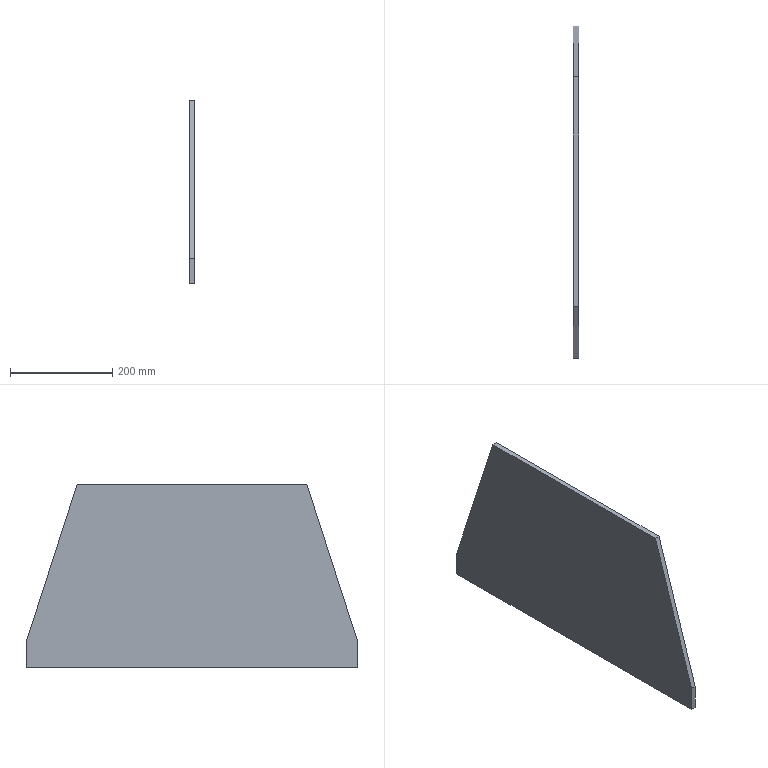Component | SolidWorks | Main-1_650X450X360X10-1 | 1 solid | 8 faces | box 10 x 650 x 360 mm | volume 2030000 mm3 | plane 8 | material Plain Carbon Steel
STEP:
#1=CARTESIAN_POINT('',(-132.764,88.438,207.322));
#2=VERTEX_POINT('',#1);
#3=CARTESIAN_POINT('',(-132.764,84.501,219.527));
#4=VERTEX_POINT('',#3);
#5=CARTESIAN_POINT('',(-132.764,84.501,219.527));
#6=DIRECTION('',(0.,-0.307,0.9517));
#7=VECTOR('',#6,39.37);
#8=LINE('',#5,#7);
#9=EDGE_CURVE('',#2,#4,#8,.T.);
#10=ORIENTED_EDGE('',*,*,#9,.F.);
#11=CARTESIAN_POINT('',(-133.157,88.438,207.322));
#12=VERTEX_POINT('',#11);
#13=CARTESIAN_POINT('',(-133.157,88.438,207.322));
#14=DIRECTION('',(1.,0.,-0.));
#15=VECTOR('',#14,39.37);
#16=LINE('',#13,#15);
#17=EDGE_CURVE('',#12,#2,#16,.T.);
#18=ORIENTED_EDGE('',*,*,#17,.F.);
#19=CARTESIAN_POINT('',(-133.157,84.501,219.527));
#20=VERTEX_POINT('',#19);
#21=CARTESIAN_POINT('',(-133.157,84.501,219.527));
#22=DIRECTION('',(0.,-0.307,0.9517));
#23=VECTOR('',#22,39.37);
#24=LINE('',#21,#23);
#25=EDGE_CURVE('',#12,#20,#24,.T.);
#26=ORIENTED_EDGE('',*,*,#25,.T.);
#27=CARTESIAN_POINT('',(-133.157,84.501,219.527));
#28=DIRECTION('',(1.,0.,-0.));
#29=VECTOR('',#28,39.37);
#30=LINE('',#27,#29);
#31=EDGE_CURVE('',#20,#4,#30,.T.);
#32=ORIENTED_EDGE('',*,*,#31,.T.);
#33=EDGE_LOOP('',(#10,#18,#26,#32));
#34=FACE_OUTER_BOUND('',#33,.T.);
#35=CARTESIAN_POINT('',(-133.157,84.501,219.527));
#36=DIRECTION('',(-0.,0.9517,0.307));
#37=DIRECTION('',(0.,-0.307,0.9517));
#38=AXIS2_PLACEMENT_3D('',#35,#36,#37);
#39=PLANE('',#38);
#40=ADVANCED_FACE('',(#34),#39,.T.);
#41=CARTESIAN_POINT('',(-132.764,88.438,205.353));
#42=VERTEX_POINT('',#41);
#43=CARTESIAN_POINT('',(-132.764,88.438,207.322));
#44=DIRECTION('',(0.,-0.,1.));
#45=VECTOR('',#44,39.37);
#46=LINE('',#43,#45);
#47=EDGE_CURVE('',#42,#2,#46,.T.);
#48=ORIENTED_EDGE('',*,*,#47,.F.);
#49=CARTESIAN_POINT('',(-133.157,88.438,205.353));
#50=VERTEX_POINT('',#49);
#51=CARTESIAN_POINT('',(-133.157,88.438,205.353));
#52=DIRECTION('',(1.,0.,-0.));
#53=VECTOR('',#52,39.37);
#54=LINE('',#51,#53);
#55=EDGE_CURVE('',#50,#42,#54,.T.);
#56=ORIENTED_EDGE('',*,*,#55,.F.);
#57=CARTESIAN_POINT('',(-133.157,88.438,207.322));
#58=DIRECTION('',(0.,-0.,1.));
#59=VECTOR('',#58,39.37);
#60=LINE('',#57,#59);
#61=EDGE_CURVE('',#50,#12,#60,.T.);
#62=ORIENTED_EDGE('',*,*,#61,.T.);
#63=ORIENTED_EDGE('',*,*,#17,.T.);
#64=EDGE_LOOP('',(#48,#56,#62,#63));
#65=FACE_OUTER_BOUND('',#64,.T.);
#66=CARTESIAN_POINT('',(-133.157,88.438,207.322));
#67=DIRECTION('',(-0.,1.,0.));
#68=DIRECTION('',(0.,-0.,1.));
#69=AXIS2_PLACEMENT_3D('',#66,#67,#68);
#70=PLANE('',#69);
#71=ADVANCED_FACE('',(#65),#70,.T.);
#72=CARTESIAN_POINT('',(-132.764,62.847,205.353));
#73=VERTEX_POINT('',#72);
#74=CARTESIAN_POINT('',(-132.764,88.438,205.353));
#75=DIRECTION('',(-0.,1.,0.));
#76=VECTOR('',#75,39.37);
#77=LINE('',#74,#76);
#78=EDGE_CURVE('',#73,#42,#77,.T.);
#79=ORIENTED_EDGE('',*,*,#78,.F.);
#80=CARTESIAN_POINT('',(-133.157,62.847,205.353));
#81=VERTEX_POINT('',#80);
#82=CARTESIAN_POINT('',(-133.157,62.847,205.353));
#83=DIRECTION('',(1.,0.,-0.));
#84=VECTOR('',#83,39.37);
#85=LINE('',#82,#84);
#86=EDGE_CURVE('',#81,#73,#85,.T.);
#87=ORIENTED_EDGE('',*,*,#86,.F.);
#88=CARTESIAN_POINT('',(-133.157,88.438,205.353));
#89=DIRECTION('',(-0.,1.,0.));
#90=VECTOR('',#89,39.37);
#91=LINE('',#88,#90);
#92=EDGE_CURVE('',#81,#50,#91,.T.);
#93=ORIENTED_EDGE('',*,*,#92,.T.);
#94=ORIENTED_EDGE('',*,*,#55,.T.);
#95=EDGE_LOOP('',(#79,#87,#93,#94));
#96=FACE_OUTER_BOUND('',#95,.T.);
#97=CARTESIAN_POINT('',(-133.157,88.438,205.353));
#98=DIRECTION('',(-0.,0.,-1.));
#99=DIRECTION('',(-0.,1.,0.));
#100=AXIS2_PLACEMENT_3D('',#97,#98,#99);
#101=PLANE('',#100);
#102=ADVANCED_FACE('',(#96),#101,.T.);
#103=CARTESIAN_POINT('',(-132.764,62.847,207.322));
#104=VERTEX_POINT('',#103);
#105=CARTESIAN_POINT('',(-132.764,62.847,205.353));
#106=DIRECTION('',(-0.,0.,-1.));
#107=VECTOR('',#106,39.37);
#108=LINE('',#105,#107);
#109=EDGE_CURVE('',#104,#73,#108,.T.);
#110=ORIENTED_EDGE('',*,*,#109,.F.);
#111=CARTESIAN_POINT('',(-133.157,62.847,207.322));
#112=VERTEX_POINT('',#111);
#113=CARTESIAN_POINT('',(-133.157,62.847,207.322));
#114=DIRECTION('',(1.,0.,-0.));
#115=VECTOR('',#114,39.37);
#116=LINE('',#113,#115);
#117=EDGE_CURVE('',#112,#104,#116,.T.);
#118=ORIENTED_EDGE('',*,*,#117,.F.);
#119=CARTESIAN_POINT('',(-133.157,62.847,205.353));
#120=DIRECTION('',(-0.,0.,-1.));
#121=VECTOR('',#120,39.37);
#122=LINE('',#119,#121);
#123=EDGE_CURVE('',#112,#81,#122,.T.);
#124=ORIENTED_EDGE('',*,*,#123,.T.);
#125=ORIENTED_EDGE('',*,*,#86,.T.);
#126=EDGE_LOOP('',(#110,#118,#124,#125));
#127=FACE_OUTER_BOUND('',#126,.T.);
#128=CARTESIAN_POINT('',(-133.157,62.847,205.353));
#129=DIRECTION('',(0.,-1.,-0.));
#130=DIRECTION('',(-0.,0.,-1.));
#131=AXIS2_PLACEMENT_3D('',#128,#129,#130);
#132=PLANE('',#131);
#133=ADVANCED_FACE('',(#127),#132,.T.);
#134=CARTESIAN_POINT('',(-132.764,66.784,219.527));
#135=VERTEX_POINT('',#134);
#136=CARTESIAN_POINT('',(-132.764,62.847,207.322));
#137=DIRECTION('',(-0.,-0.307,-0.9517));
#138=VECTOR('',#137,39.37);
#139=LINE('',#136,#138);
#140=EDGE_CURVE('',#135,#104,#139,.T.);
#141=ORIENTED_EDGE('',*,*,#140,.F.);
#142=CARTESIAN_POINT('',(-133.157,66.784,219.527));
#143=VERTEX_POINT('',#142);
#144=CARTESIAN_POINT('',(-133.157,66.784,219.527));
#145=DIRECTION('',(1.,0.,-0.));
#146=VECTOR('',#145,39.37);
#147=LINE('',#144,#146);
#148=EDGE_CURVE('',#143,#135,#147,.T.);
#149=ORIENTED_EDGE('',*,*,#148,.F.);
#150=CARTESIAN_POINT('',(-133.157,62.847,207.322));
#151=DIRECTION('',(-0.,-0.307,-0.9517));
#152=VECTOR('',#151,39.37);
#153=LINE('',#150,#152);
#154=EDGE_CURVE('',#143,#112,#153,.T.);
#155=ORIENTED_EDGE('',*,*,#154,.T.);
#156=ORIENTED_EDGE('',*,*,#117,.T.);
#157=EDGE_LOOP('',(#141,#149,#155,#156));
#158=FACE_OUTER_BOUND('',#157,.T.);
#159=CARTESIAN_POINT('',(-133.157,62.847,207.322));
#160=DIRECTION('',(0.,-0.9517,0.307));
#161=DIRECTION('',(-0.,-0.307,-0.9517));
#162=AXIS2_PLACEMENT_3D('',#159,#160,#161);
#163=PLANE('',#162);
#164=ADVANCED_FACE('',(#158),#163,.T.);
#165=CARTESIAN_POINT('',(-132.764,66.784,219.527));
#166=DIRECTION('',(0.,-1.,-0.));
#167=VECTOR('',#166,39.37);
#168=LINE('',#165,#167);
#169=EDGE_CURVE('',#4,#135,#168,.T.);
#170=ORIENTED_EDGE('',*,*,#169,.F.);
#171=ORIENTED_EDGE('',*,*,#31,.F.);
#172=CARTESIAN_POINT('',(-133.157,66.784,219.527));
#173=DIRECTION('',(0.,-1.,-0.));
#174=VECTOR('',#173,39.37);
#175=LINE('',#172,#174);
#176=EDGE_CURVE('',#20,#143,#175,.T.);
#177=ORIENTED_EDGE('',*,*,#176,.T.);
#178=ORIENTED_EDGE('',*,*,#148,.T.);
#179=EDGE_LOOP('',(#170,#171,#177,#178));
#180=FACE_OUTER_BOUND('',#179,.T.);
#181=CARTESIAN_POINT('',(-133.157,66.784,219.527));
#182=DIRECTION('',(0.,-0.,1.));
#183=DIRECTION('',(0.,-1.,-0.));
#184=AXIS2_PLACEMENT_3D('',#181,#182,#183);
#185=PLANE('',#184);
#186=ADVANCED_FACE('',(#180),#185,.T.);
#187=ORIENTED_EDGE('',*,*,#25,.F.);
#188=ORIENTED_EDGE('',*,*,#61,.F.);
#189=ORIENTED_EDGE('',*,*,#92,.F.);
#190=ORIENTED_EDGE('',*,*,#123,.F.);
#191=ORIENTED_EDGE('',*,*,#154,.F.);
#192=ORIENTED_EDGE('',*,*,#176,.F.);
#193=EDGE_LOOP('',(#187,#188,#189,#190,#191,#192));
#194=FACE_OUTER_BOUND('',#193,.T.);
#195=CARTESIAN_POINT('',(-133.157,62.847,219.527));
#196=DIRECTION('',(-1.,-0.,0.));
#197=DIRECTION('',(0.,-0.,1.));
#198=AXIS2_PLACEMENT_3D('',#195,#196,#197);
#199=PLANE('',#198);
#200=ADVANCED_FACE('',(#194),#199,.T.);
#201=ORIENTED_EDGE('',*,*,#9,.T.);
#202=ORIENTED_EDGE('',*,*,#169,.T.);
#203=ORIENTED_EDGE('',*,*,#140,.T.);
#204=ORIENTED_EDGE('',*,*,#109,.T.);
#205=ORIENTED_EDGE('',*,*,#78,.T.);
#206=ORIENTED_EDGE('',*,*,#47,.T.);
#207=EDGE_LOOP('',(#201,#202,#203,#204,#205,#206));
#208=FACE_OUTER_BOUND('',#207,.T.);
#209=CARTESIAN_POINT('',(-132.764,62.847,219.527));
#210=DIRECTION('',(-1.,-0.,0.));
#211=DIRECTION('',(0.,-0.,1.));
#212=AXIS2_PLACEMENT_3D('',#209,#210,#211);
#213=PLANE('',#212);
#214=ADVANCED_FACE('',(#208),#213,.F.);
#215=CLOSED_SHELL('',(#40,#71,#102,#133,#164,#186,#200,#214));
#216=MANIFOLD_SOLID_BREP('',#215);
#217=CARTESIAN_POINT('',(0.,0.,0.));
#218=DIRECTION('',(0.,0.,1.));
#219=DIRECTION('',(1.,0.,0.));
#220=AXIS2_PLACEMENT_3D('',#217,#218,#219);
#221=(LENGTH_UNIT()NAMED_UNIT(*)SI_UNIT($,.METRE.));
#222=LENGTH_MEASURE_WITH_UNIT(LENGTH_MEASURE(0.0254),#221);
#223=DIMENSIONAL_EXPONENTS(1.,0.,0.,0.,0.,0.,0.);
#224=(CONVERSION_BASED_UNIT('',#222)LENGTH_UNIT()NAMED_UNIT(#223));
#225=UNCERTAINTY_MEASURE_WITH_UNIT(LENGTH_MEASURE(0.00001),#224,'','');
#226=(NAMED_UNIT(*)PLANE_ANGLE_UNIT()SI_UNIT($,.RADIAN.));
#227=(NAMED_UNIT(*)SI_UNIT($,.STERADIAN.)SOLID_ANGLE_UNIT());
#228=(GEOMETRIC_REPRESENTATION_CONTEXT(3)GLOBAL_UNCERTAINTY_ASSIGNED_CONTEXT((#225))GLOBAL_UNIT_ASSIGNED_CONTEXT((#224,#226,#227))REPRESENTATION_CONTEXT('',''));
#229=ADVANCED_BREP_SHAPE_REPRESENTATION('',(#216,#220),#228);
#230=COLOUR_RGB('',0.7922,0.8196,0.9333);
#231=FILL_AREA_STYLE_COLOUR('',#230);
#232=FILL_AREA_STYLE('',(#231));
#233=SURFACE_STYLE_FILL_AREA(#232);
#234=SURFACE_SIDE_STYLE('',(#233));
#235=SURFACE_STYLE_USAGE(.BOTH.,#234);
#236=PRESENTATION_STYLE_ASSIGNMENT((#235));
#237=STYLED_ITEM('',(#236),#216);
#238=(LENGTH_UNIT()NAMED_UNIT(*)SI_UNIT($,.METRE.));
#239=LENGTH_MEASURE_WITH_UNIT(LENGTH_MEASURE(0.0254),#238);
#240=DIMENSIONAL_EXPONENTS(1.,0.,0.,0.,0.,0.,0.);
#241=(CONVERSION_BASED_UNIT('',#239)LENGTH_UNIT()NAMED_UNIT(#240));
#242=UNCERTAINTY_MEASURE_WITH_UNIT(LENGTH_MEASURE(0.00001),#241,'','');
#243=(NAMED_UNIT(*)PLANE_ANGLE_UNIT()SI_UNIT($,.RADIAN.));
#244=(NAMED_UNIT(*)SI_UNIT($,.STERADIAN.)SOLID_ANGLE_UNIT());
#245=(GEOMETRIC_REPRESENTATION_CONTEXT(3)GLOBAL_UNCERTAINTY_ASSIGNED_CONTEXT((#242))GLOBAL_UNIT_ASSIGNED_CONTEXT((#241,#243,#244))REPRESENTATION_CONTEXT('',''));
#246=MECHANICAL_DESIGN_GEOMETRIC_PRESENTATION_REPRESENTATION('',(#237),#245);
#247=PRESENTATION_LAYER_ASSIGNMENT('','',(#237));